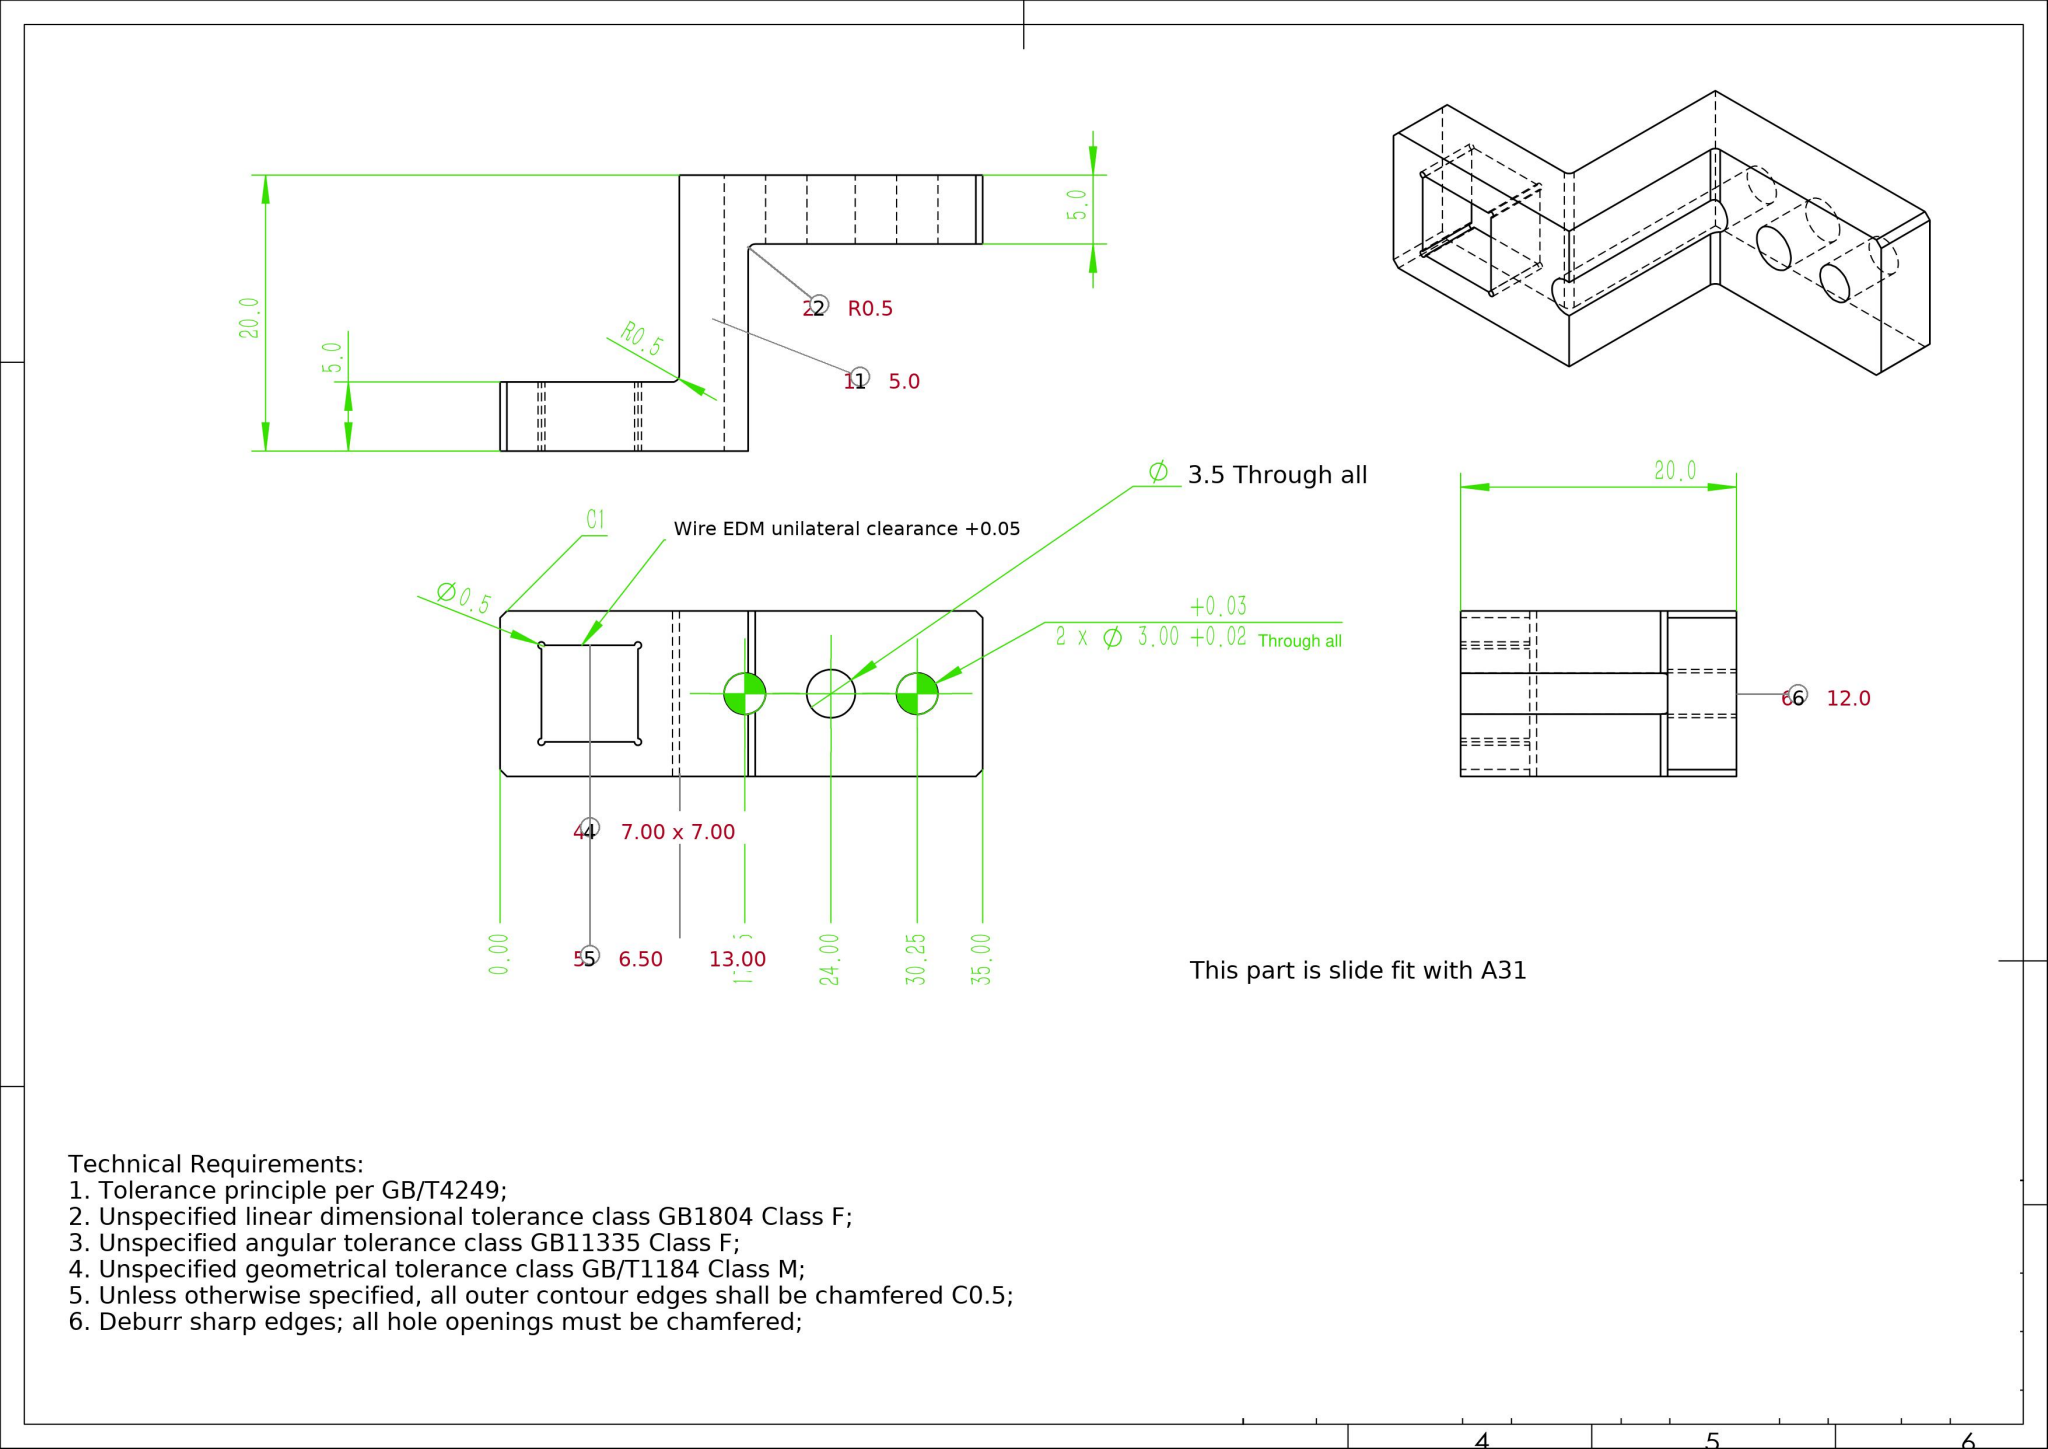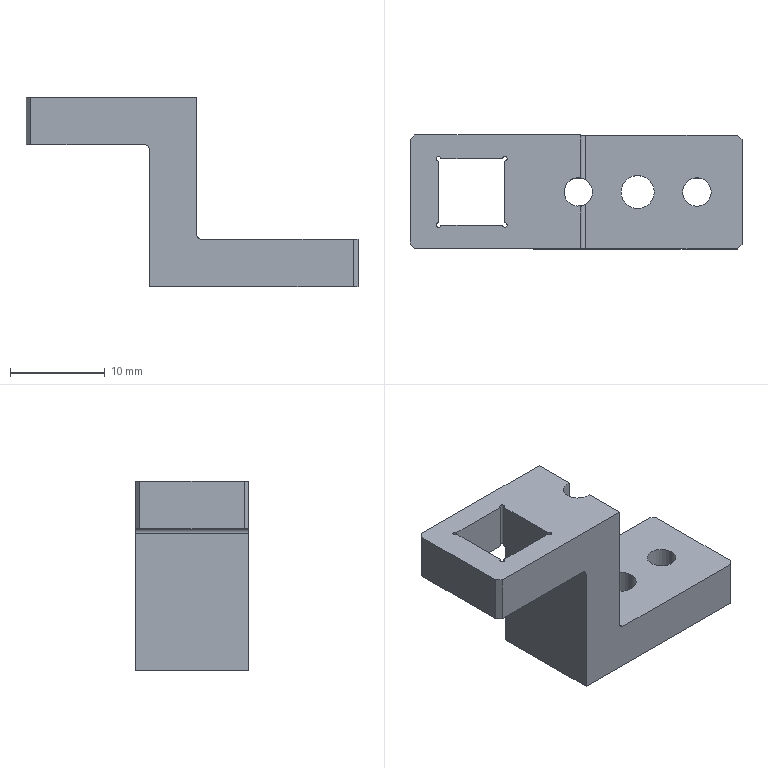Part | SolidWorks | mm | 1 solid | 34 faces | box 35 x 12 x 20 mm | volume 2568 mm3 | plane 19 | cylinder 15 | commonest cylinder face diameters 0.5 x6 3 x4 1 x3 3.5 x2
build123d program:
from build123d import *

# Parameters (mm, degrees)
SKETCH1_W                  = 35
SKETCH1_H                  = 12
BOSS_EXTRUDE1_DEPTH        = 20
CUT_EXTRUDE1_DEPTH         = 28.244
CUT_EXTRUDE1_DEPTH_BACK    = 28.244
SKETCH2_W                  = 7
SKETCH2_H                  = 7
SKETCH3_W                  = 17
SKETCH3_H                  = 12
CUT_EXTRUDE2_DEPTH         = 15
SKETCH4_W                  = 13
SKETCH4_H                  = 15
CUT_EXTRUDE3_DEPTH         = 30.159
SIZE_MM_DOWEL_PIN_HOLE2_D  = 1.5
F_3_5_3_5_DIAMETER_HOLE1_D = 3.5
F_0_5_0_5_DIAMETER_HOLE1_D = 0.5
FILLET1_R                  = 0.5
CHAMFER1_SIZE              = 0.5
CHAMFER2_SIZE              = 0.5
SIZE_MM_DOWEL_PIN_HOLE3_D  = 3


with BuildPart() as part:
    # Sketch1 → Boss-Extrude1 (new body)
    with BuildSketch(Plane.XY):
        Rectangle(SKETCH1_W, SKETCH1_H)
    extrude(amount=BOSS_EXTRUDE1_DEPTH)

    # Sketch2 → Cut-Extrude1 (cut, two sides: drawn at the far end of the back side and taken through both)
    with BuildSketch(Plane.XY.offset(20).offset(-CUT_EXTRUDE1_DEPTH_BACK)):
        with Locations((-11, 0)):
            Rectangle(SKETCH2_W, SKETCH2_H)
    extrude(amount=CUT_EXTRUDE1_DEPTH + CUT_EXTRUDE1_DEPTH_BACK, mode=Mode.SUBTRACT)

    # Sketch3 → Cut-Extrude2 (cut)
    with BuildSketch(Plane.XY.offset(20)):
        with Locations((9, 0)):
            Rectangle(SKETCH3_W, SKETCH3_H)
    extrude(amount=-CUT_EXTRUDE2_DEPTH, mode=Mode.SUBTRACT)

    # Sketch4 → Cut-Extrude3 (cut, through all)
    with BuildSketch(Plane.XZ.offset(6)):
        with Locations((-11, 7.5)):
            Rectangle(SKETCH4_W, SKETCH4_H)
    extrude(amount=-CUT_EXTRUDE3_DEPTH, mode=Mode.SUBTRACT)

    # Size mm Dowel Pin Hole2 (through all)
    with Locations(Plane(origin=(0, 0, 0), x_dir=(-1, 0, 0), z_dir=(0, 0, -1))):
        with Locations((-6.5, 0)):
            Hole(SIZE_MM_DOWEL_PIN_HOLE2_D / 2)

    # 3.5 _3.5_ Diameter Hole1 (through all)
    with Locations(Plane.XY.offset(5)):
        with Locations((6.5, 0)):
            Hole(F_3_5_3_5_DIAMETER_HOLE1_D / 2)

    # 0.5 _0.5_ Diameter Hole1 (through all)
    with Locations(Plane.XY.offset(20)):
        with Locations((-14.5, 3.5), (-7.5, 3.5), (-14.5, -3.5), (-7.5, -3.5)):
            Hole(F_0_5_0_5_DIAMETER_HOLE1_D / 2)

    # Fillet1
    fillet1_edges = [part.edges().sort_by_distance(p)[0] for p in [
        (0.5, 0, 5),
        (-4.5, 0, 15),
    ]]
    fillet(fillet1_edges, radius=FILLET1_R)

    # Chamfer1
    chamfer1_edges = [part.edges().sort_by_distance(p)[0] for p in [
        (-17.5, 6, 17.5),
        (-17.5, -6, 17.5),
    ]]
    chamfer(chamfer1_edges, length=CHAMFER1_SIZE)

    # Chamfer2
    chamfer2_edges = [part.edges().sort_by_distance(p)[0] for p in [
        (17.5, 6, 2.5),
        (17.5, -6, 2.5),
    ]]
    chamfer(chamfer2_edges, length=CHAMFER2_SIZE)

    # Size mm Dowel Pin Hole3 (through all)
    with Locations(Plane(origin=(0, 0, 0), x_dir=(-1, 0, 0), z_dir=(0, 0, -1))):
        with Locations((-0.25, 0), (-12.75, 0)):
            Hole(SIZE_MM_DOWEL_PIN_HOLE3_D / 2)


solid = part.part